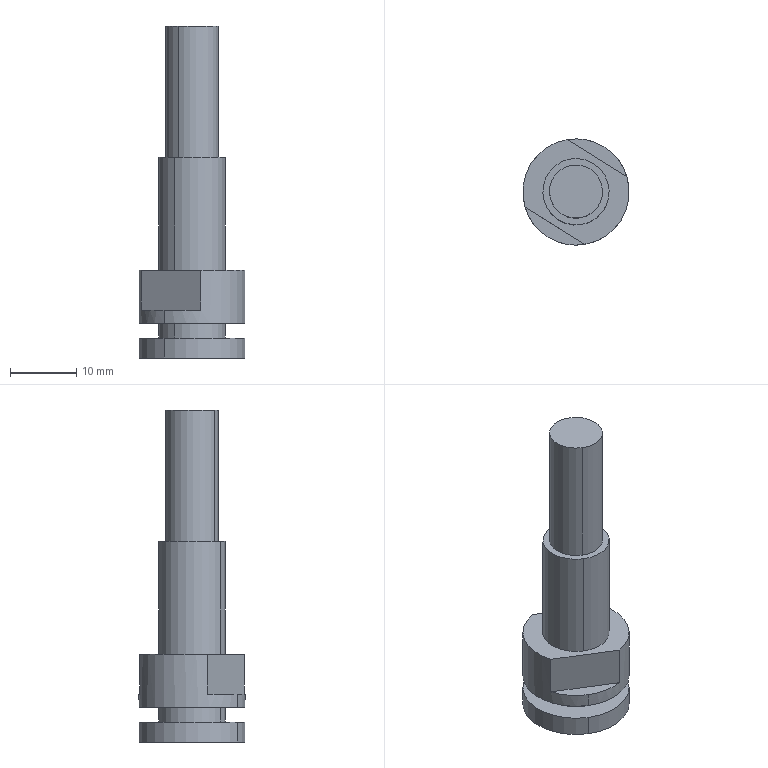Component | SolidWorks | DirectPressureVerticalSeal-1_ThrustStud-1 | 1 solid | 20 faces | box 16 x 16 x 50 mm | volume 4541 mm3 | cylinder 10 | plane 10 | commonest cylinder face diameters 10 x4 16 x4 8 x2
build123d program:
from build123d import *

# Parameters (mm, degrees)
CUT_EXTRUDE1_DEPTH  = 6
CUT_EXTRUDE2_DEPTH  = 6
BOSS_EXTRUDE1_START = 17
SKETCH4_R           = 5
BOSS_EXTRUDE1_DEPTH = 17
SKETCH5_R           = 4
BOSS_EXTRUDE2_DEPTH = 19.8


with BuildPart() as part:
    # Sketch1 → Revolve1 (revolve)
    with BuildSketch(Plane(origin=(0, 0, 0), x_dir=(-1, 0, 0), z_dir=(0, 0, -1)), mode=Mode.PRIVATE) as revolve1_sk:
        Polygon((-13.2, 8), (-13.2, 0), (0, 0), (0, 8), (-3, 8), (-3, 5), (-5.2, 5), (-5.2, 8), align=None)
    revolve(revolve1_sk.sketch.rotate(Axis((13.2, 0, 0), (-1, 0, 0)), 270), axis=Axis((13.2, 0, 0), (-1, 0, 0)))

    # Sketch2 → Cut-Extrude1 (cut)
    with BuildSketch(Plane(origin=(13.2, 0, 0), x_dir=(0, 0, -1), z_dir=(1, 0, 0))):
        with BuildLine():
            Line((-6, -5.292), (-6, 5.292))
            ThreePointArc((-6, 5.292), (-8, 0), (-6, -5.292))
        make_face()
    extrude(amount=-CUT_EXTRUDE1_DEPTH, mode=Mode.SUBTRACT)

    # Sketch3 → Cut-Extrude2 (cut)
    with BuildSketch(Plane(origin=(13.2, 0, 0), x_dir=(0, 0, -1), z_dir=(1, 0, 0))):
        with BuildLine():
            Line((6, 5.292), (6, -5.292))
            ThreePointArc((6, -5.292), (8, 0), (6, 5.292))
        make_face()
    extrude(amount=-CUT_EXTRUDE2_DEPTH, mode=Mode.SUBTRACT)

    # Sketch4 → Boss-Extrude1 (add)
    with BuildSketch(Plane(origin=(13.2, 0, 0), x_dir=(0, 0, -1), z_dir=(1, 0, 0)).offset(BOSS_EXTRUDE1_START)):
        with Locations(Location((0, 0, 0), (0, 0, 180))):
            Circle(SKETCH4_R)
    extrude(amount=-BOSS_EXTRUDE1_DEPTH)

    # Sketch5 → Boss-Extrude2 (add)
    with BuildSketch(Plane(origin=(30.2, 0, 0), x_dir=(0, 0, -1), z_dir=(1, 0, 0))):
        Circle(SKETCH5_R)
    extrude(amount=BOSS_EXTRUDE2_DEPTH)


solid = part.part

# Placed as in the assembly
solid = solid.moved(Location((-298.746, 246.873, 258.854), (-90, 31.792, -90)))
STEP:
#1=COLOUR_RGB('',0.7922,0.8196,0.9333);
#2=FILL_AREA_STYLE_COLOUR('',#1);
#3=FILL_AREA_STYLE('',(#2));
#4=SURFACE_STYLE_FILL_AREA(#3);
#5=SURFACE_SIDE_STYLE('',(#4));
#6=SURFACE_STYLE_USAGE(.BOTH.,#5);
#7=PRESENTATION_STYLE_ASSIGNMENT((#6));
#8=CARTESIAN_POINT('',(-11.679,9.853,12.16));
#9=VERTEX_POINT('',#8);
#10=CARTESIAN_POINT('',(-11.845,9.586,12.16));
#11=VERTEX_POINT('',#10);
#12=CARTESIAN_POINT('',(-11.762,9.719,12.16));
#13=DIRECTION('',(-0.,0.,1.));
#14=DIRECTION('',(0.5268,0.85,0.));
#15=AXIS2_PLACEMENT_3D('',#12,#13,#14);
#16=CIRCLE('',#15,0.1575);
#17=EDGE_CURVE('',#9,#11,#16,.T.);
#18=ORIENTED_EDGE('',*,*,#17,.F.);
#19=CARTESIAN_POINT('',(-11.679,9.853,11.38));
#20=VERTEX_POINT('',#19);
#21=CARTESIAN_POINT('',(-11.679,9.853,12.16));
#22=DIRECTION('',(0.,-0.,-1.));
#23=VECTOR('',#22,39.37);
#24=LINE('',#21,#23);
#25=EDGE_CURVE('',#9,#20,#24,.T.);
#26=ORIENTED_EDGE('',*,*,#25,.T.);
#27=CARTESIAN_POINT('',(-11.845,9.586,11.38));
#28=VERTEX_POINT('',#27);
#29=CARTESIAN_POINT('',(-11.762,9.719,11.38));
#30=DIRECTION('',(-0.,0.,1.));
#31=DIRECTION('',(0.5268,0.85,0.));
#32=AXIS2_PLACEMENT_3D('',#29,#30,#31);
#33=CIRCLE('',#32,0.1575);
#34=EDGE_CURVE('',#20,#28,#33,.T.);
#35=ORIENTED_EDGE('',*,*,#34,.T.);
#36=CARTESIAN_POINT('',(-11.845,9.586,12.16));
#37=DIRECTION('',(0.,-0.,-1.));
#38=VECTOR('',#37,39.37);
#39=LINE('',#36,#38);
#40=EDGE_CURVE('',#11,#28,#39,.T.);
#41=ORIENTED_EDGE('',*,*,#40,.F.);
#42=EDGE_LOOP('',(#18,#26,#35,#41));
#43=FACE_OUTER_BOUND('',#42,.T.);
#44=CARTESIAN_POINT('',(-11.762,9.719,12.16));
#45=DIRECTION('',(0.,-0.,-1.));
#46=DIRECTION('',(-0.5268,-0.85,0.));
#47=AXIS2_PLACEMENT_3D('',#44,#45,#46);
#48=CYLINDRICAL_SURFACE('',#47,0.1575);
#49=ADVANCED_FACE('',(#43),#48,.T.);
#50=CARTESIAN_POINT('',(-11.658,9.887,11.38));
#51=VERTEX_POINT('',#50);
#52=CARTESIAN_POINT('',(-11.865,9.552,11.38));
#53=VERTEX_POINT('',#52);
#54=CARTESIAN_POINT('',(-11.762,9.719,11.38));
#55=DIRECTION('',(-0.,0.,1.));
#56=DIRECTION('',(0.5268,0.85,0.));
#57=AXIS2_PLACEMENT_3D('',#54,#55,#56);
#58=CIRCLE('',#57,0.1969);
#59=EDGE_CURVE('',#51,#53,#58,.T.);
#60=ORIENTED_EDGE('',*,*,#59,.F.);
#61=CARTESIAN_POINT('',(-11.658,9.887,10.711));
#62=VERTEX_POINT('',#61);
#63=CARTESIAN_POINT('',(-11.658,9.887,11.38));
#64=DIRECTION('',(0.,-0.,-1.));
#65=VECTOR('',#64,39.37);
#66=LINE('',#63,#65);
#67=EDGE_CURVE('',#51,#62,#66,.T.);
#68=ORIENTED_EDGE('',*,*,#67,.T.);
#69=CARTESIAN_POINT('',(-11.865,9.552,10.711));
#70=VERTEX_POINT('',#69);
#71=CARTESIAN_POINT('',(-11.762,9.719,10.711));
#72=DIRECTION('',(-0.,0.,1.));
#73=DIRECTION('',(0.5268,0.85,0.));
#74=AXIS2_PLACEMENT_3D('',#71,#72,#73);
#75=CIRCLE('',#74,0.1969);
#76=EDGE_CURVE('',#62,#70,#75,.T.);
#77=ORIENTED_EDGE('',*,*,#76,.T.);
#78=CARTESIAN_POINT('',(-11.865,9.552,11.38));
#79=DIRECTION('',(0.,-0.,-1.));
#80=VECTOR('',#79,39.37);
#81=LINE('',#78,#80);
#82=EDGE_CURVE('',#53,#70,#81,.T.);
#83=ORIENTED_EDGE('',*,*,#82,.F.);
#84=EDGE_LOOP('',(#60,#68,#77,#83));
#85=FACE_OUTER_BOUND('',#84,.T.);
#86=CARTESIAN_POINT('',(-11.762,9.719,11.38));
#87=DIRECTION('',(0.,-0.,-1.));
#88=DIRECTION('',(-0.5268,-0.85,0.));
#89=AXIS2_PLACEMENT_3D('',#86,#87,#88);
#90=CYLINDRICAL_SURFACE('',#89,0.1969);
#91=ADVANCED_FACE('',(#85),#90,.T.);
#92=CARTESIAN_POINT('',(-11.865,9.552,10.396));
#93=VERTEX_POINT('',#92);
#94=CARTESIAN_POINT('',(-11.658,9.887,10.396));
#95=VERTEX_POINT('',#94);
#96=CARTESIAN_POINT('',(-11.762,9.719,10.396));
#97=DIRECTION('',(0.,-0.,-1.));
#98=DIRECTION('',(-0.5268,-0.85,0.));
#99=AXIS2_PLACEMENT_3D('',#96,#97,#98);
#100=CIRCLE('',#99,0.1969);
#101=EDGE_CURVE('',#93,#95,#100,.T.);
#102=ORIENTED_EDGE('',*,*,#101,.T.);
#103=CARTESIAN_POINT('',(-11.658,9.887,10.309));
#104=VERTEX_POINT('',#103);
#105=CARTESIAN_POINT('',(-11.658,9.887,10.711));
#106=DIRECTION('',(0.,-0.,-1.));
#107=VECTOR('',#106,39.37);
#108=LINE('',#105,#107);
#109=EDGE_CURVE('',#95,#104,#108,.T.);
#110=ORIENTED_EDGE('',*,*,#109,.T.);
#111=CARTESIAN_POINT('',(-11.865,9.552,10.309));
#112=VERTEX_POINT('',#111);
#113=CARTESIAN_POINT('',(-11.762,9.719,10.309));
#114=DIRECTION('',(0.,-0.,-1.));
#115=DIRECTION('',(-0.5268,-0.85,0.));
#116=AXIS2_PLACEMENT_3D('',#113,#114,#115);
#117=CIRCLE('',#116,0.1969);
#118=EDGE_CURVE('',#112,#104,#117,.T.);
#119=ORIENTED_EDGE('',*,*,#118,.F.);
#120=CARTESIAN_POINT('',(-11.865,9.552,10.711));
#121=DIRECTION('',(0.,-0.,-1.));
#122=VECTOR('',#121,39.37);
#123=LINE('',#120,#122);
#124=EDGE_CURVE('',#93,#112,#123,.T.);
#125=ORIENTED_EDGE('',*,*,#124,.F.);
#126=EDGE_LOOP('',(#102,#110,#119,#125));
#127=FACE_OUTER_BOUND('',#126,.T.);
#128=CARTESIAN_POINT('',(-11.762,9.719,10.711));
#129=DIRECTION('',(0.,-0.,-1.));
#130=DIRECTION('',(-0.5268,-0.85,0.));
#131=AXIS2_PLACEMENT_3D('',#128,#129,#130);
#132=CYLINDRICAL_SURFACE('',#131,0.1969);
#133=ADVANCED_FACE('',(#127),#132,.T.);
#134=CARTESIAN_POINT('',(-11.928,9.452,10.309));
#135=VERTEX_POINT('',#134);
#136=CARTESIAN_POINT('',(-11.596,9.987,10.309));
#137=VERTEX_POINT('',#136);
#138=CARTESIAN_POINT('',(-11.762,9.719,10.309));
#139=DIRECTION('',(0.,-0.,-1.));
#140=DIRECTION('',(-0.5268,-0.85,0.));
#141=AXIS2_PLACEMENT_3D('',#138,#139,#140);
#142=CIRCLE('',#141,0.315);
#143=EDGE_CURVE('',#135,#137,#142,.T.);
#144=ORIENTED_EDGE('',*,*,#143,.T.);
#145=CARTESIAN_POINT('',(-11.596,9.987,10.191));
#146=VERTEX_POINT('',#145);
#147=CARTESIAN_POINT('',(-11.596,9.987,10.711));
#148=DIRECTION('',(0.,-0.,-1.));
#149=VECTOR('',#148,39.37);
#150=LINE('',#147,#149);
#151=EDGE_CURVE('',#137,#146,#150,.T.);
#152=ORIENTED_EDGE('',*,*,#151,.T.);
#153=CARTESIAN_POINT('',(-11.928,9.452,10.191));
#154=VERTEX_POINT('',#153);
#155=CARTESIAN_POINT('',(-11.762,9.719,10.191));
#156=DIRECTION('',(0.,-0.,-1.));
#157=DIRECTION('',(-0.5268,-0.85,0.));
#158=AXIS2_PLACEMENT_3D('',#155,#156,#157);
#159=CIRCLE('',#158,0.315);
#160=EDGE_CURVE('',#154,#146,#159,.T.);
#161=ORIENTED_EDGE('',*,*,#160,.F.);
#162=CARTESIAN_POINT('',(-11.928,9.452,10.711));
#163=DIRECTION('',(0.,-0.,-1.));
#164=VECTOR('',#163,39.37);
#165=LINE('',#162,#164);
#166=EDGE_CURVE('',#135,#154,#165,.T.);
#167=ORIENTED_EDGE('',*,*,#166,.F.);
#168=EDGE_LOOP('',(#144,#152,#161,#167));
#169=FACE_OUTER_BOUND('',#168,.T.);
#170=CARTESIAN_POINT('',(-11.762,9.719,10.711));
#171=DIRECTION('',(0.,-0.,-1.));
#172=DIRECTION('',(-0.5268,-0.85,0.));
#173=AXIS2_PLACEMENT_3D('',#170,#171,#172);
#174=CYLINDRICAL_SURFACE('',#173,0.315);
#175=ADVANCED_FACE('',(#169),#174,.T.);
#176=CARTESIAN_POINT('',(-11.596,9.987,10.475));
#177=VERTEX_POINT('',#176);
#178=CARTESIAN_POINT('',(-11.814,10.03,10.475));
#179=VERTEX_POINT('',#178);
#180=CARTESIAN_POINT('',(-11.762,9.719,10.475));
#181=DIRECTION('',(-0.,0.,1.));
#182=DIRECTION('',(0.5268,0.85,0.));
#183=AXIS2_PLACEMENT_3D('',#180,#181,#182);
#184=CIRCLE('',#183,0.315);
#185=EDGE_CURVE('',#177,#179,#184,.T.);
#186=ORIENTED_EDGE('',*,*,#185,.F.);
#187=CARTESIAN_POINT('',(-11.596,9.987,10.396));
#188=VERTEX_POINT('',#187);
#189=CARTESIAN_POINT('',(-11.596,9.987,10.711));
#190=DIRECTION('',(0.,-0.,-1.));
#191=VECTOR('',#190,39.37);
#192=LINE('',#189,#191);
#193=EDGE_CURVE('',#177,#188,#192,.T.);
#194=ORIENTED_EDGE('',*,*,#193,.T.);
#195=CARTESIAN_POINT('',(-11.928,9.452,10.396));
#196=VERTEX_POINT('',#195);
#197=CARTESIAN_POINT('',(-11.762,9.719,10.396));
#198=DIRECTION('',(0.,-0.,-1.));
#199=DIRECTION('',(-0.5268,-0.85,0.));
#200=AXIS2_PLACEMENT_3D('',#197,#198,#199);
#201=CIRCLE('',#200,0.315);
#202=EDGE_CURVE('',#196,#188,#201,.T.);
#203=ORIENTED_EDGE('',*,*,#202,.F.);
#204=CARTESIAN_POINT('',(-11.928,9.452,10.475));
#205=VERTEX_POINT('',#204);
#206=CARTESIAN_POINT('',(-11.928,9.452,10.711));
#207=DIRECTION('',(0.,-0.,-1.));
#208=VECTOR('',#207,39.37);
#209=LINE('',#206,#208);
#210=EDGE_CURVE('',#205,#196,#209,.T.);
#211=ORIENTED_EDGE('',*,*,#210,.F.);
#212=CARTESIAN_POINT('',(-12.063,9.628,10.475));
#213=VERTEX_POINT('',#212);
#214=CARTESIAN_POINT('',(-11.762,9.719,10.475));
#215=DIRECTION('',(-0.,0.,1.));
#216=DIRECTION('',(0.5268,0.85,0.));
#217=AXIS2_PLACEMENT_3D('',#214,#215,#216);
#218=CIRCLE('',#217,0.315);
#219=EDGE_CURVE('',#213,#205,#218,.T.);
#220=ORIENTED_EDGE('',*,*,#219,.F.);
#221=CARTESIAN_POINT('',(-12.063,9.628,10.711));
#222=VERTEX_POINT('',#221);
#223=CARTESIAN_POINT('',(-12.063,9.628,10.475));
#224=DIRECTION('',(-0.,0.,1.));
#225=VECTOR('',#224,39.37);
#226=LINE('',#223,#225);
#227=EDGE_CURVE('',#213,#222,#226,.T.);
#228=ORIENTED_EDGE('',*,*,#227,.T.);
#229=CARTESIAN_POINT('',(-11.814,10.03,10.711));
#230=VERTEX_POINT('',#229);
#231=CARTESIAN_POINT('',(-11.762,9.719,10.711));
#232=DIRECTION('',(0.,-0.,-1.));
#233=DIRECTION('',(-0.5268,-0.85,0.));
#234=AXIS2_PLACEMENT_3D('',#231,#232,#233);
#235=CIRCLE('',#234,0.315);
#236=EDGE_CURVE('',#222,#230,#235,.T.);
#237=ORIENTED_EDGE('',*,*,#236,.T.);
#238=CARTESIAN_POINT('',(-11.814,10.03,10.475));
#239=DIRECTION('',(-0.,0.,1.));
#240=VECTOR('',#239,39.37);
#241=LINE('',#238,#240);
#242=EDGE_CURVE('',#179,#230,#241,.T.);
#243=ORIENTED_EDGE('',*,*,#242,.F.);
#244=EDGE_LOOP('',(#186,#194,#203,#211,#220,#228,#237,#243));
#245=FACE_OUTER_BOUND('',#244,.T.);
#246=CARTESIAN_POINT('',(-11.762,9.719,10.711));
#247=DIRECTION('',(0.,-0.,-1.));
#248=DIRECTION('',(-0.5268,-0.85,0.));
#249=AXIS2_PLACEMENT_3D('',#246,#247,#248);
#250=CYLINDRICAL_SURFACE('',#249,0.315);
#251=ADVANCED_FACE('',(#245),#250,.T.);
#252=ORIENTED_EDGE('',*,*,#193,.F.);
#253=CARTESIAN_POINT('',(-11.46,9.81,10.475));
#254=VERTEX_POINT('',#253);
#255=CARTESIAN_POINT('',(-11.762,9.719,10.475));
#256=DIRECTION('',(-0.,0.,1.));
#257=DIRECTION('',(0.5268,0.85,0.));
#258=AXIS2_PLACEMENT_3D('',#255,#256,#257);
#259=CIRCLE('',#258,0.315);
#260=EDGE_CURVE('',#254,#177,#259,.T.);
#261=ORIENTED_EDGE('',*,*,#260,.F.);
#262=CARTESIAN_POINT('',(-11.46,9.81,10.711));
#263=VERTEX_POINT('',#262);
#264=CARTESIAN_POINT('',(-11.46,9.81,10.475));
#265=DIRECTION('',(-0.,0.,1.));
#266=VECTOR('',#265,39.37);
#267=LINE('',#264,#266);
#268=EDGE_CURVE('',#254,#263,#267,.T.);
#269=ORIENTED_EDGE('',*,*,#268,.T.);
#270=CARTESIAN_POINT('',(-11.709,9.409,10.711));
#271=VERTEX_POINT('',#270);
#272=CARTESIAN_POINT('',(-11.762,9.719,10.711));
#273=DIRECTION('',(0.,-0.,-1.));
#274=DIRECTION('',(-0.5268,-0.85,0.));
#275=AXIS2_PLACEMENT_3D('',#272,#273,#274);
#276=CIRCLE('',#275,0.315);
#277=EDGE_CURVE('',#263,#271,#276,.T.);
#278=ORIENTED_EDGE('',*,*,#277,.T.);
#279=CARTESIAN_POINT('',(-11.709,9.409,10.475));
#280=VERTEX_POINT('',#279);
#281=CARTESIAN_POINT('',(-11.709,9.409,10.475));
#282=DIRECTION('',(-0.,0.,1.));
#283=VECTOR('',#282,39.37);
#284=LINE('',#281,#283);
#285=EDGE_CURVE('',#280,#271,#284,.T.);
#286=ORIENTED_EDGE('',*,*,#285,.F.);
#287=CARTESIAN_POINT('',(-11.762,9.719,10.475));
#288=DIRECTION('',(-0.,0.,1.));
#289=DIRECTION('',(0.5268,0.85,0.));
#290=AXIS2_PLACEMENT_3D('',#287,#288,#289);
#291=CIRCLE('',#290,0.315);
#292=EDGE_CURVE('',#205,#280,#291,.T.);
#293=ORIENTED_EDGE('',*,*,#292,.F.);
#294=ORIENTED_EDGE('',*,*,#210,.T.);
#295=CARTESIAN_POINT('',(-11.762,9.719,10.396));
#296=DIRECTION('',(0.,-0.,-1.));
#297=DIRECTION('',(-0.5268,-0.85,0.));
#298=AXIS2_PLACEMENT_3D('',#295,#296,#297);
#299=CIRCLE('',#298,0.315);
#300=EDGE_CURVE('',#188,#196,#299,.T.);
#301=ORIENTED_EDGE('',*,*,#300,.F.);
#302=EDGE_LOOP('',(#252,#261,#269,#278,#286,#293,#294,#301));
#303=FACE_OUTER_BOUND('',#302,.T.);
#304=CARTESIAN_POINT('',(-11.762,9.719,10.711));
#305=DIRECTION('',(0.,-0.,-1.));
#306=DIRECTION('',(-0.5268,-0.85,0.));
#307=AXIS2_PLACEMENT_3D('',#304,#305,#306);
#308=CYLINDRICAL_SURFACE('',#307,0.315);
#309=ADVANCED_FACE('',(#303),#308,.T.);
#310=CARTESIAN_POINT('',(-11.762,9.719,10.711));
#311=DIRECTION('',(-0.,0.,1.));
#312=DIRECTION('',(0.5268,0.85,0.));
#313=AXIS2_PLACEMENT_3D('',#310,#311,#312);
#314=CIRCLE('',#313,0.1969);
#315=EDGE_CURVE('',#70,#62,#314,.T.);
#316=ORIENTED_EDGE('',*,*,#315,.F.);
#317=ORIENTED_EDGE('',*,*,#76,.F.);
#318=EDGE_LOOP('',(#316,#317));
#319=FACE_BOUND('',#318,.T.);
#320=CARTESIAN_POINT('',(-11.814,10.03,10.711));
#321=DIRECTION('',(0.85,-0.5268,0.));
#322=VECTOR('',#321,39.37);
#323=LINE('',#320,#322);
#324=EDGE_CURVE('',#230,#263,#323,.T.);
#325=ORIENTED_EDGE('',*,*,#324,.F.);
#326=ORIENTED_EDGE('',*,*,#236,.F.);
#327=CARTESIAN_POINT('',(-11.709,9.409,10.711));
#328=DIRECTION('',(-0.85,0.5268,-0.));
#329=VECTOR('',#328,39.37);
#330=LINE('',#327,#329);
#331=EDGE_CURVE('',#271,#222,#330,.T.);
#332=ORIENTED_EDGE('',*,*,#331,.F.);
#333=ORIENTED_EDGE('',*,*,#277,.F.);
#334=EDGE_LOOP('',(#325,#326,#332,#333));
#335=FACE_OUTER_BOUND('',#334,.T.);
#336=CARTESIAN_POINT('',(-12.029,9.885,10.711));
#337=DIRECTION('',(-0.,0.,1.));
#338=DIRECTION('',(0.5268,0.85,0.));
#339=AXIS2_PLACEMENT_3D('',#336,#337,#338);
#340=PLANE('',#339);
#341=ADVANCED_FACE('',(#319,#335),#340,.T.);
#342=ORIENTED_EDGE('',*,*,#160,.T.);
#343=CARTESIAN_POINT('',(-11.762,9.719,10.191));
#344=DIRECTION('',(0.,-0.,-1.));
#345=DIRECTION('',(-0.5268,-0.85,0.));
#346=AXIS2_PLACEMENT_3D('',#343,#344,#345);
#347=CIRCLE('',#346,0.315);
#348=EDGE_CURVE('',#146,#154,#347,.T.);
#349=ORIENTED_EDGE('',*,*,#348,.T.);
#350=EDGE_LOOP('',(#342,#349));
#351=FACE_OUTER_BOUND('',#350,.T.);
#352=CARTESIAN_POINT('',(-11.762,9.719,10.191));
#353=DIRECTION('',(0.,-0.,-1.));
#354=DIRECTION('',(-0.5268,-0.85,-0.));
#355=AXIS2_PLACEMENT_3D('',#352,#353,#354);
#356=PLANE('',#355);
#357=ADVANCED_FACE('',(#351),#356,.T.);
#358=ORIENTED_EDGE('',*,*,#151,.F.);
#359=CARTESIAN_POINT('',(-11.762,9.719,10.309));
#360=DIRECTION('',(0.,-0.,-1.));
#361=DIRECTION('',(-0.5268,-0.85,0.));
#362=AXIS2_PLACEMENT_3D('',#359,#360,#361);
#363=CIRCLE('',#362,0.315);
#364=EDGE_CURVE('',#137,#135,#363,.T.);
#365=ORIENTED_EDGE('',*,*,#364,.T.);
#366=ORIENTED_EDGE('',*,*,#166,.T.);
#367=ORIENTED_EDGE('',*,*,#348,.F.);
#368=EDGE_LOOP('',(#358,#365,#366,#367));
#369=FACE_OUTER_BOUND('',#368,.T.);
#370=CARTESIAN_POINT('',(-11.762,9.719,10.711));
#371=DIRECTION('',(0.,-0.,-1.));
#372=DIRECTION('',(-0.5268,-0.85,0.));
#373=AXIS2_PLACEMENT_3D('',#370,#371,#372);
#374=CYLINDRICAL_SURFACE('',#373,0.315);
#375=ADVANCED_FACE('',(#369),#374,.T.);
#376=ORIENTED_EDGE('',*,*,#118,.T.);
#377=CARTESIAN_POINT('',(-11.762,9.719,10.309));
#378=DIRECTION('',(0.,-0.,-1.));
#379=DIRECTION('',(-0.5268,-0.85,0.));
#380=AXIS2_PLACEMENT_3D('',#377,#378,#379);
#381=CIRCLE('',#380,0.1969);
#382=EDGE_CURVE('',#104,#112,#381,.T.);
#383=ORIENTED_EDGE('',*,*,#382,.T.);
#384=EDGE_LOOP('',(#376,#383));
#385=FACE_BOUND('',#384,.T.);
#386=ORIENTED_EDGE('',*,*,#143,.F.);
#387=ORIENTED_EDGE('',*,*,#364,.F.);
#388=EDGE_LOOP('',(#386,#387));
#389=FACE_OUTER_BOUND('',#388,.T.);
#390=CARTESIAN_POINT('',(-12.029,9.885,10.309));
#391=DIRECTION('',(-0.,0.,1.));
#392=DIRECTION('',(0.5268,0.85,0.));
#393=AXIS2_PLACEMENT_3D('',#390,#391,#392);
#394=PLANE('',#393);
#395=ADVANCED_FACE('',(#385,#389),#394,.T.);
#396=ORIENTED_EDGE('',*,*,#109,.F.);
#397=CARTESIAN_POINT('',(-11.762,9.719,10.396));
#398=DIRECTION('',(0.,-0.,-1.));
#399=DIRECTION('',(-0.5268,-0.85,0.));
#400=AXIS2_PLACEMENT_3D('',#397,#398,#399);
#401=CIRCLE('',#400,0.1969);
#402=EDGE_CURVE('',#95,#93,#401,.T.);
#403=ORIENTED_EDGE('',*,*,#402,.T.);
#404=ORIENTED_EDGE('',*,*,#124,.T.);
#405=ORIENTED_EDGE('',*,*,#382,.F.);
#406=EDGE_LOOP('',(#396,#403,#404,#405));
#407=FACE_OUTER_BOUND('',#406,.T.);
#408=CARTESIAN_POINT('',(-11.762,9.719,10.711));
#409=DIRECTION('',(0.,-0.,-1.));
#410=DIRECTION('',(-0.5268,-0.85,0.));
#411=AXIS2_PLACEMENT_3D('',#408,#409,#410);
#412=CYLINDRICAL_SURFACE('',#411,0.1969);
#413=ADVANCED_FACE('',(#407),#412,.T.);
#414=ORIENTED_EDGE('',*,*,#202,.T.);
#415=ORIENTED_EDGE('',*,*,#300,.T.);
#416=EDGE_LOOP('',(#414,#415));
#417=FACE_OUTER_BOUND('',#416,.T.);
#418=ORIENTED_EDGE('',*,*,#101,.F.);
#419=ORIENTED_EDGE('',*,*,#402,.F.);
#420=EDGE_LOOP('',(#418,#419));
#421=FACE_BOUND('',#420,.T.);
#422=CARTESIAN_POINT('',(-11.929,9.823,10.396));
#423=DIRECTION('',(0.,-0.,-1.));
#424=DIRECTION('',(-0.5268,-0.85,-0.));
#425=AXIS2_PLACEMENT_3D('',#422,#423,#424);
#426=PLANE('',#425);
#427=ADVANCED_FACE('',(#417,#421),#426,.T.);
#428=ORIENTED_EDGE('',*,*,#331,.T.);
#429=ORIENTED_EDGE('',*,*,#227,.F.);
#430=CARTESIAN_POINT('',(-11.709,9.409,10.475));
#431=DIRECTION('',(-0.85,0.5268,-0.));
#432=VECTOR('',#431,39.37);
#433=LINE('',#430,#432);
#434=EDGE_CURVE('',#280,#213,#433,.T.);
#435=ORIENTED_EDGE('',*,*,#434,.F.);
#436=ORIENTED_EDGE('',*,*,#285,.T.);
#437=EDGE_LOOP('',(#428,#429,#435,#436));
#438=FACE_OUTER_BOUND('',#437,.T.);
#439=CARTESIAN_POINT('',(-11.709,9.409,10.475));
#440=DIRECTION('',(0.5268,0.85,0.));
#441=DIRECTION('',(0.,-0.,-1.));
#442=AXIS2_PLACEMENT_3D('',#439,#440,#441);
#443=PLANE('',#442);
#444=ADVANCED_FACE('',(#438),#443,.F.);
#445=ORIENTED_EDGE('',*,*,#219,.T.);
#446=ORIENTED_EDGE('',*,*,#292,.T.);
#447=ORIENTED_EDGE('',*,*,#434,.T.);
#448=EDGE_LOOP('',(#445,#446,#447));
#449=FACE_OUTER_BOUND('',#448,.T.);
#450=CARTESIAN_POINT('',(-11.762,9.719,10.475));
#451=DIRECTION('',(-0.,0.,1.));
#452=DIRECTION('',(0.5268,0.85,0.));
#453=AXIS2_PLACEMENT_3D('',#450,#451,#452);
#454=PLANE('',#453);
#455=ADVANCED_FACE('',(#449),#454,.T.);
#456=ORIENTED_EDGE('',*,*,#324,.T.);
#457=ORIENTED_EDGE('',*,*,#268,.F.);
#458=CARTESIAN_POINT('',(-11.814,10.03,10.475));
#459=DIRECTION('',(0.85,-0.5268,0.));
#460=VECTOR('',#459,39.37);
#461=LINE('',#458,#460);
#462=EDGE_CURVE('',#179,#254,#461,.T.);
#463=ORIENTED_EDGE('',*,*,#462,.F.);
#464=ORIENTED_EDGE('',*,*,#242,.T.);
#465=EDGE_LOOP('',(#456,#457,#463,#464));
#466=FACE_OUTER_BOUND('',#465,.T.);
#467=CARTESIAN_POINT('',(-11.814,10.03,10.475));
#468=DIRECTION('',(-0.5268,-0.85,-0.));
#469=DIRECTION('',(-0.,0.,1.));
#470=AXIS2_PLACEMENT_3D('',#467,#468,#469);
#471=PLANE('',#470);
#472=ADVANCED_FACE('',(#466),#471,.F.);
#473=ORIENTED_EDGE('',*,*,#260,.T.);
#474=ORIENTED_EDGE('',*,*,#185,.T.);
#475=ORIENTED_EDGE('',*,*,#462,.T.);
#476=EDGE_LOOP('',(#473,#474,#475));
#477=FACE_OUTER_BOUND('',#476,.T.);
#478=CARTESIAN_POINT('',(-11.762,9.719,10.475));
#479=DIRECTION('',(-0.,0.,1.));
#480=DIRECTION('',(0.5268,0.85,0.));
#481=AXIS2_PLACEMENT_3D('',#478,#479,#480);
#482=PLANE('',#481);
#483=ADVANCED_FACE('',(#477),#482,.T.);
#484=ORIENTED_EDGE('',*,*,#67,.F.);
#485=CARTESIAN_POINT('',(-11.762,9.719,11.38));
#486=DIRECTION('',(-0.,0.,1.));
#487=DIRECTION('',(0.5268,0.85,0.));
#488=AXIS2_PLACEMENT_3D('',#485,#486,#487);
#489=CIRCLE('',#488,0.1969);
#490=EDGE_CURVE('',#53,#51,#489,.T.);
#491=ORIENTED_EDGE('',*,*,#490,.F.);
#492=ORIENTED_EDGE('',*,*,#82,.T.);
#493=ORIENTED_EDGE('',*,*,#315,.T.);
#494=EDGE_LOOP('',(#484,#491,#492,#493));
#495=FACE_OUTER_BOUND('',#494,.T.);
#496=CARTESIAN_POINT('',(-11.762,9.719,11.38));
#497=DIRECTION('',(0.,-0.,-1.));
#498=DIRECTION('',(-0.5268,-0.85,0.));
#499=AXIS2_PLACEMENT_3D('',#496,#497,#498);
#500=CYLINDRICAL_SURFACE('',#499,0.1969);
#501=ADVANCED_FACE('',(#495),#500,.T.);
#502=CARTESIAN_POINT('',(-11.762,9.719,11.38));
#503=DIRECTION('',(-0.,0.,1.));
#504=DIRECTION('',(0.5268,0.85,0.));
#505=AXIS2_PLACEMENT_3D('',#502,#503,#504);
#506=CIRCLE('',#505,0.1575);
#507=EDGE_CURVE('',#28,#20,#506,.T.);
#508=ORIENTED_EDGE('',*,*,#507,.F.);
#509=ORIENTED_EDGE('',*,*,#34,.F.);
#510=EDGE_LOOP('',(#508,#509));
#511=FACE_BOUND('',#510,.T.);
#512=ORIENTED_EDGE('',*,*,#490,.T.);
#513=ORIENTED_EDGE('',*,*,#59,.T.);
#514=EDGE_LOOP('',(#512,#513));
#515=FACE_OUTER_BOUND('',#514,.T.);
#516=CARTESIAN_POINT('',(-11.762,9.719,11.38));
#517=DIRECTION('',(-0.,0.,1.));
#518=DIRECTION('',(0.5268,0.85,0.));
#519=AXIS2_PLACEMENT_3D('',#516,#517,#518);
#520=PLANE('',#519);
#521=ADVANCED_FACE('',(#511,#515),#520,.T.);
#522=ORIENTED_EDGE('',*,*,#25,.F.);
#523=CARTESIAN_POINT('',(-11.762,9.719,12.16));
#524=DIRECTION('',(-0.,0.,1.));
#525=DIRECTION('',(0.5268,0.85,0.));
#526=AXIS2_PLACEMENT_3D('',#523,#524,#525);
#527=CIRCLE('',#526,0.1575);
#528=EDGE_CURVE('',#11,#9,#527,.T.);
#529=ORIENTED_EDGE('',*,*,#528,.F.);
#530=ORIENTED_EDGE('',*,*,#40,.T.);
#531=ORIENTED_EDGE('',*,*,#507,.T.);
#532=EDGE_LOOP('',(#522,#529,#530,#531));
#533=FACE_OUTER_BOUND('',#532,.T.);
#534=CARTESIAN_POINT('',(-11.762,9.719,12.16));
#535=DIRECTION('',(0.,-0.,-1.));
#536=DIRECTION('',(-0.5268,-0.85,0.));
#537=AXIS2_PLACEMENT_3D('',#534,#535,#536);
#538=CYLINDRICAL_SURFACE('',#537,0.1575);
#539=ADVANCED_FACE('',(#533),#538,.T.);
#540=ORIENTED_EDGE('',*,*,#528,.T.);
#541=ORIENTED_EDGE('',*,*,#17,.T.);
#542=EDGE_LOOP('',(#540,#541));
#543=FACE_OUTER_BOUND('',#542,.T.);
#544=CARTESIAN_POINT('',(-11.762,9.719,12.16));
#545=DIRECTION('',(-0.,0.,1.));
#546=DIRECTION('',(0.5268,0.85,0.));
#547=AXIS2_PLACEMENT_3D('',#544,#545,#546);
#548=PLANE('',#547);
#549=ADVANCED_FACE('',(#543),#548,.T.);
#550=CLOSED_SHELL('',(#49,#91,#133,#175,#251,#309,#341,#357,#375,#395,#413,#427,#444,#455,#472,#483,#501,#521,#539,#549));
#551=MANIFOLD_SOLID_BREP('',#550);
#552=STYLED_ITEM('',(#7),#551);
#553=PRESENTATION_LAYER_ASSIGNMENT('','',(#552));
#554=CARTESIAN_POINT('',(0.,0.,0.));
#555=DIRECTION('',(0.,0.,1.));
#556=DIRECTION('',(1.,0.,0.));
#557=AXIS2_PLACEMENT_3D('',#554,#555,#556);
#558=(LENGTH_UNIT()NAMED_UNIT(*)SI_UNIT($,.METRE.));
#559=LENGTH_MEASURE_WITH_UNIT(LENGTH_MEASURE(0.0254),#558);
#560=DIMENSIONAL_EXPONENTS(1.,0.,0.,0.,0.,0.,0.);
#561=(CONVERSION_BASED_UNIT('',#559)LENGTH_UNIT()NAMED_UNIT(#560));
#562=UNCERTAINTY_MEASURE_WITH_UNIT(LENGTH_MEASURE(0.00001),#561,'','');
#563=(NAMED_UNIT(*)PLANE_ANGLE_UNIT()SI_UNIT($,.RADIAN.));
#564=(NAMED_UNIT(*)SI_UNIT($,.STERADIAN.)SOLID_ANGLE_UNIT());
#565=(GEOMETRIC_REPRESENTATION_CONTEXT(3)GLOBAL_UNCERTAINTY_ASSIGNED_CONTEXT((#562))GLOBAL_UNIT_ASSIGNED_CONTEXT((#561,#563,#564))REPRESENTATION_CONTEXT('',''));
#566=ADVANCED_BREP_SHAPE_REPRESENTATION('',(#551,#557),#565);
#567=(LENGTH_UNIT()NAMED_UNIT(*)SI_UNIT($,.METRE.));
#568=LENGTH_MEASURE_WITH_UNIT(LENGTH_MEASURE(0.0254),#567);
#569=DIMENSIONAL_EXPONENTS(1.,0.,0.,0.,0.,0.,0.);
#570=(CONVERSION_BASED_UNIT('',#568)LENGTH_UNIT()NAMED_UNIT(#569));
#571=UNCERTAINTY_MEASURE_WITH_UNIT(LENGTH_MEASURE(0.00001),#570,'','');
#572=(NAMED_UNIT(*)PLANE_ANGLE_UNIT()SI_UNIT($,.RADIAN.));
#573=(NAMED_UNIT(*)SI_UNIT($,.STERADIAN.)SOLID_ANGLE_UNIT());
#574=(GEOMETRIC_REPRESENTATION_CONTEXT(3)GLOBAL_UNCERTAINTY_ASSIGNED_CONTEXT((#571))GLOBAL_UNIT_ASSIGNED_CONTEXT((#570,#572,#573))REPRESENTATION_CONTEXT('',''));
#575=MECHANICAL_DESIGN_GEOMETRIC_PRESENTATION_REPRESENTATION('',(#552),#574);